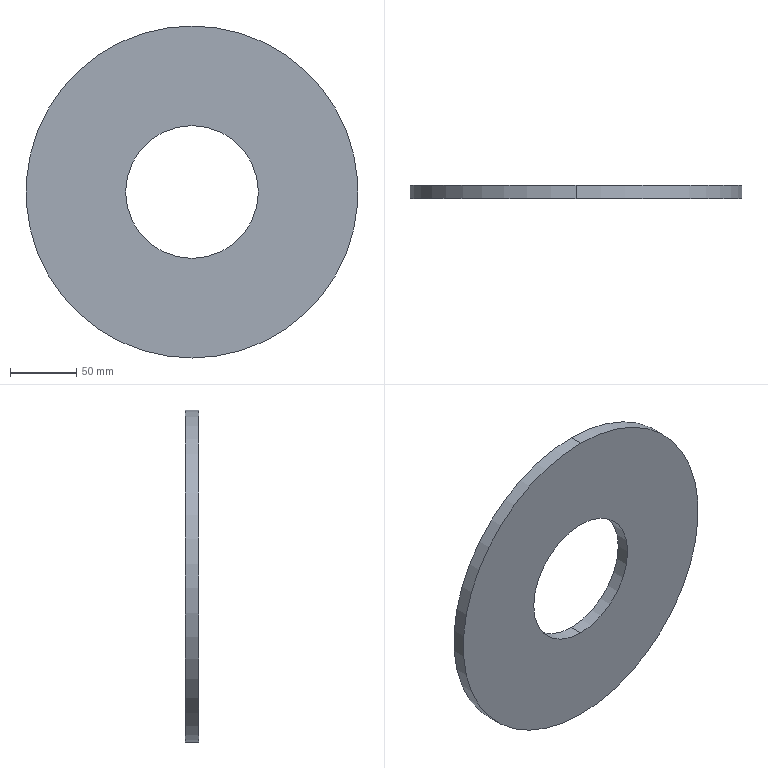Component | SolidWorks | Support3-1 | 1 solid | 6 faces | box 250 x 10 x 250 mm | volume 412334 mm3 | cylinder 4 | plane 2 | commonest cylinder face diameters 100 x2 250 x2 | material Plain Carbon Steel
STEP:
#1=COLOUR_RGB('',0.7922,0.8196,0.9333);
#2=FILL_AREA_STYLE_COLOUR('',#1);
#3=FILL_AREA_STYLE('',(#2));
#4=SURFACE_STYLE_FILL_AREA(#3);
#5=SURFACE_SIDE_STYLE('',(#4));
#6=SURFACE_STYLE_USAGE(.BOTH.,#5);
#7=PRESENTATION_STYLE_ASSIGNMENT((#6));
#8=CARTESIAN_POINT('',(49.235,45.014,74.925));
#9=VERTEX_POINT('',#8);
#10=CARTESIAN_POINT('',(49.235,45.014,70.988));
#11=VERTEX_POINT('',#10);
#12=CARTESIAN_POINT('',(49.235,45.014,72.956));
#13=DIRECTION('',(-0.,1.,0.));
#14=DIRECTION('',(0.,0.,-1.));
#15=AXIS2_PLACEMENT_3D('',#12,#13,#14);
#16=CIRCLE('',#15,1.969);
#17=EDGE_CURVE('',#9,#11,#16,.T.);
#18=ORIENTED_EDGE('',*,*,#17,.F.);
#19=CARTESIAN_POINT('',(49.235,45.407,74.925));
#20=VERTEX_POINT('',#19);
#21=CARTESIAN_POINT('',(49.235,45.014,74.925));
#22=DIRECTION('',(-0.,1.,0.));
#23=VECTOR('',#22,39.37);
#24=LINE('',#21,#23);
#25=EDGE_CURVE('',#9,#20,#24,.T.);
#26=ORIENTED_EDGE('',*,*,#25,.T.);
#27=CARTESIAN_POINT('',(49.235,45.407,70.988));
#28=VERTEX_POINT('',#27);
#29=CARTESIAN_POINT('',(49.235,45.407,72.956));
#30=DIRECTION('',(-0.,1.,0.));
#31=DIRECTION('',(0.,0.,-1.));
#32=AXIS2_PLACEMENT_3D('',#29,#30,#31);
#33=CIRCLE('',#32,1.969);
#34=EDGE_CURVE('',#20,#28,#33,.T.);
#35=ORIENTED_EDGE('',*,*,#34,.T.);
#36=CARTESIAN_POINT('',(49.235,45.014,70.988));
#37=DIRECTION('',(-0.,1.,0.));
#38=VECTOR('',#37,39.37);
#39=LINE('',#36,#38);
#40=EDGE_CURVE('',#11,#28,#39,.T.);
#41=ORIENTED_EDGE('',*,*,#40,.F.);
#42=EDGE_LOOP('',(#18,#26,#35,#41));
#43=FACE_OUTER_BOUND('',#42,.T.);
#44=CARTESIAN_POINT('',(49.235,45.014,72.956));
#45=DIRECTION('',(-0.,1.,0.));
#46=DIRECTION('',(0.,0.,-1.));
#47=AXIS2_PLACEMENT_3D('',#44,#45,#46);
#48=CYLINDRICAL_SURFACE('',#47,1.969);
#49=ADVANCED_FACE('',(#43),#48,.F.);
#50=CARTESIAN_POINT('',(49.235,45.014,68.035));
#51=VERTEX_POINT('',#50);
#52=CARTESIAN_POINT('',(49.235,45.014,77.877));
#53=VERTEX_POINT('',#52);
#54=CARTESIAN_POINT('',(49.235,45.014,72.956));
#55=DIRECTION('',(-0.,1.,0.));
#56=DIRECTION('',(0.,0.,-1.));
#57=AXIS2_PLACEMENT_3D('',#54,#55,#56);
#58=CIRCLE('',#57,4.921);
#59=EDGE_CURVE('',#51,#53,#58,.T.);
#60=ORIENTED_EDGE('',*,*,#59,.T.);
#61=CARTESIAN_POINT('',(49.235,45.407,77.877));
#62=VERTEX_POINT('',#61);
#63=CARTESIAN_POINT('',(49.235,45.014,77.877));
#64=DIRECTION('',(-0.,1.,0.));
#65=VECTOR('',#64,39.37);
#66=LINE('',#63,#65);
#67=EDGE_CURVE('',#53,#62,#66,.T.);
#68=ORIENTED_EDGE('',*,*,#67,.T.);
#69=CARTESIAN_POINT('',(49.235,45.407,68.035));
#70=VERTEX_POINT('',#69);
#71=CARTESIAN_POINT('',(49.235,45.407,72.956));
#72=DIRECTION('',(-0.,1.,0.));
#73=DIRECTION('',(0.,0.,-1.));
#74=AXIS2_PLACEMENT_3D('',#71,#72,#73);
#75=CIRCLE('',#74,4.921);
#76=EDGE_CURVE('',#70,#62,#75,.T.);
#77=ORIENTED_EDGE('',*,*,#76,.F.);
#78=CARTESIAN_POINT('',(49.235,45.014,68.035));
#79=DIRECTION('',(-0.,1.,0.));
#80=VECTOR('',#79,39.37);
#81=LINE('',#78,#80);
#82=EDGE_CURVE('',#51,#70,#81,.T.);
#83=ORIENTED_EDGE('',*,*,#82,.F.);
#84=EDGE_LOOP('',(#60,#68,#77,#83));
#85=FACE_OUTER_BOUND('',#84,.T.);
#86=CARTESIAN_POINT('',(49.235,45.014,72.956));
#87=DIRECTION('',(-0.,1.,0.));
#88=DIRECTION('',(0.,0.,-1.));
#89=AXIS2_PLACEMENT_3D('',#86,#87,#88);
#90=CYLINDRICAL_SURFACE('',#89,4.921);
#91=ADVANCED_FACE('',(#85),#90,.T.);
#92=ORIENTED_EDGE('',*,*,#67,.F.);
#93=CARTESIAN_POINT('',(49.235,45.014,72.956));
#94=DIRECTION('',(-0.,1.,0.));
#95=DIRECTION('',(0.,0.,-1.));
#96=AXIS2_PLACEMENT_3D('',#93,#94,#95);
#97=CIRCLE('',#96,4.921);
#98=EDGE_CURVE('',#53,#51,#97,.T.);
#99=ORIENTED_EDGE('',*,*,#98,.T.);
#100=ORIENTED_EDGE('',*,*,#82,.T.);
#101=CARTESIAN_POINT('',(49.235,45.407,72.956));
#102=DIRECTION('',(-0.,1.,0.));
#103=DIRECTION('',(0.,0.,-1.));
#104=AXIS2_PLACEMENT_3D('',#101,#102,#103);
#105=CIRCLE('',#104,4.921);
#106=EDGE_CURVE('',#62,#70,#105,.T.);
#107=ORIENTED_EDGE('',*,*,#106,.F.);
#108=EDGE_LOOP('',(#92,#99,#100,#107));
#109=FACE_OUTER_BOUND('',#108,.T.);
#110=CARTESIAN_POINT('',(49.235,45.014,72.956));
#111=DIRECTION('',(-0.,1.,0.));
#112=DIRECTION('',(0.,0.,-1.));
#113=AXIS2_PLACEMENT_3D('',#110,#111,#112);
#114=CYLINDRICAL_SURFACE('',#113,4.921);
#115=ADVANCED_FACE('',(#109),#114,.T.);
#116=CARTESIAN_POINT('',(49.235,45.014,72.956));
#117=DIRECTION('',(-0.,1.,0.));
#118=DIRECTION('',(0.,0.,-1.));
#119=AXIS2_PLACEMENT_3D('',#116,#117,#118);
#120=CIRCLE('',#119,1.969);
#121=EDGE_CURVE('',#11,#9,#120,.T.);
#122=ORIENTED_EDGE('',*,*,#121,.T.);
#123=ORIENTED_EDGE('',*,*,#17,.T.);
#124=EDGE_LOOP('',(#122,#123));
#125=FACE_BOUND('',#124,.T.);
#126=ORIENTED_EDGE('',*,*,#59,.F.);
#127=ORIENTED_EDGE('',*,*,#98,.F.);
#128=EDGE_LOOP('',(#126,#127));
#129=FACE_OUTER_BOUND('',#128,.T.);
#130=CARTESIAN_POINT('',(49.235,45.014,72.956));
#131=DIRECTION('',(-0.,1.,0.));
#132=DIRECTION('',(0.,0.,-1.));
#133=AXIS2_PLACEMENT_3D('',#130,#131,#132);
#134=PLANE('',#133);
#135=ADVANCED_FACE('',(#125,#129),#134,.F.);
#136=CARTESIAN_POINT('',(49.235,45.407,72.956));
#137=DIRECTION('',(-0.,1.,0.));
#138=DIRECTION('',(0.,0.,-1.));
#139=AXIS2_PLACEMENT_3D('',#136,#137,#138);
#140=CIRCLE('',#139,1.969);
#141=EDGE_CURVE('',#28,#20,#140,.T.);
#142=ORIENTED_EDGE('',*,*,#141,.F.);
#143=ORIENTED_EDGE('',*,*,#34,.F.);
#144=EDGE_LOOP('',(#142,#143));
#145=FACE_BOUND('',#144,.T.);
#146=ORIENTED_EDGE('',*,*,#76,.T.);
#147=ORIENTED_EDGE('',*,*,#106,.T.);
#148=EDGE_LOOP('',(#146,#147));
#149=FACE_OUTER_BOUND('',#148,.T.);
#150=CARTESIAN_POINT('',(49.235,45.407,72.956));
#151=DIRECTION('',(-0.,1.,0.));
#152=DIRECTION('',(0.,0.,-1.));
#153=AXIS2_PLACEMENT_3D('',#150,#151,#152);
#154=PLANE('',#153);
#155=ADVANCED_FACE('',(#145,#149),#154,.T.);
#156=ORIENTED_EDGE('',*,*,#25,.F.);
#157=ORIENTED_EDGE('',*,*,#121,.F.);
#158=ORIENTED_EDGE('',*,*,#40,.T.);
#159=ORIENTED_EDGE('',*,*,#141,.T.);
#160=EDGE_LOOP('',(#156,#157,#158,#159));
#161=FACE_OUTER_BOUND('',#160,.T.);
#162=CARTESIAN_POINT('',(49.235,45.014,72.956));
#163=DIRECTION('',(-0.,1.,0.));
#164=DIRECTION('',(0.,0.,-1.));
#165=AXIS2_PLACEMENT_3D('',#162,#163,#164);
#166=CYLINDRICAL_SURFACE('',#165,1.969);
#167=ADVANCED_FACE('',(#161),#166,.F.);
#168=CLOSED_SHELL('',(#49,#91,#115,#135,#155,#167));
#169=MANIFOLD_SOLID_BREP('',#168);
#170=STYLED_ITEM('',(#7),#169);
#171=PRESENTATION_LAYER_ASSIGNMENT('','',(#170));
#172=CARTESIAN_POINT('',(0.,0.,0.));
#173=DIRECTION('',(0.,0.,1.));
#174=DIRECTION('',(1.,0.,0.));
#175=AXIS2_PLACEMENT_3D('',#172,#173,#174);
#176=(LENGTH_UNIT()NAMED_UNIT(*)SI_UNIT($,.METRE.));
#177=LENGTH_MEASURE_WITH_UNIT(LENGTH_MEASURE(0.0254),#176);
#178=DIMENSIONAL_EXPONENTS(1.,0.,0.,0.,0.,0.,0.);
#179=(CONVERSION_BASED_UNIT('',#177)LENGTH_UNIT()NAMED_UNIT(#178));
#180=UNCERTAINTY_MEASURE_WITH_UNIT(LENGTH_MEASURE(0.00001),#179,'','');
#181=(NAMED_UNIT(*)PLANE_ANGLE_UNIT()SI_UNIT($,.RADIAN.));
#182=(NAMED_UNIT(*)SI_UNIT($,.STERADIAN.)SOLID_ANGLE_UNIT());
#183=(GEOMETRIC_REPRESENTATION_CONTEXT(3)GLOBAL_UNCERTAINTY_ASSIGNED_CONTEXT((#180))GLOBAL_UNIT_ASSIGNED_CONTEXT((#179,#181,#182))REPRESENTATION_CONTEXT('',''));
#184=ADVANCED_BREP_SHAPE_REPRESENTATION('',(#169,#175),#183);
#185=(LENGTH_UNIT()NAMED_UNIT(*)SI_UNIT($,.METRE.));
#186=LENGTH_MEASURE_WITH_UNIT(LENGTH_MEASURE(0.0254),#185);
#187=DIMENSIONAL_EXPONENTS(1.,0.,0.,0.,0.,0.,0.);
#188=(CONVERSION_BASED_UNIT('',#186)LENGTH_UNIT()NAMED_UNIT(#187));
#189=UNCERTAINTY_MEASURE_WITH_UNIT(LENGTH_MEASURE(0.00001),#188,'','');
#190=(NAMED_UNIT(*)PLANE_ANGLE_UNIT()SI_UNIT($,.RADIAN.));
#191=(NAMED_UNIT(*)SI_UNIT($,.STERADIAN.)SOLID_ANGLE_UNIT());
#192=(GEOMETRIC_REPRESENTATION_CONTEXT(3)GLOBAL_UNCERTAINTY_ASSIGNED_CONTEXT((#189))GLOBAL_UNIT_ASSIGNED_CONTEXT((#188,#190,#191))REPRESENTATION_CONTEXT('',''));
#193=MECHANICAL_DESIGN_GEOMETRIC_PRESENTATION_REPRESENTATION('',(#170),#192);